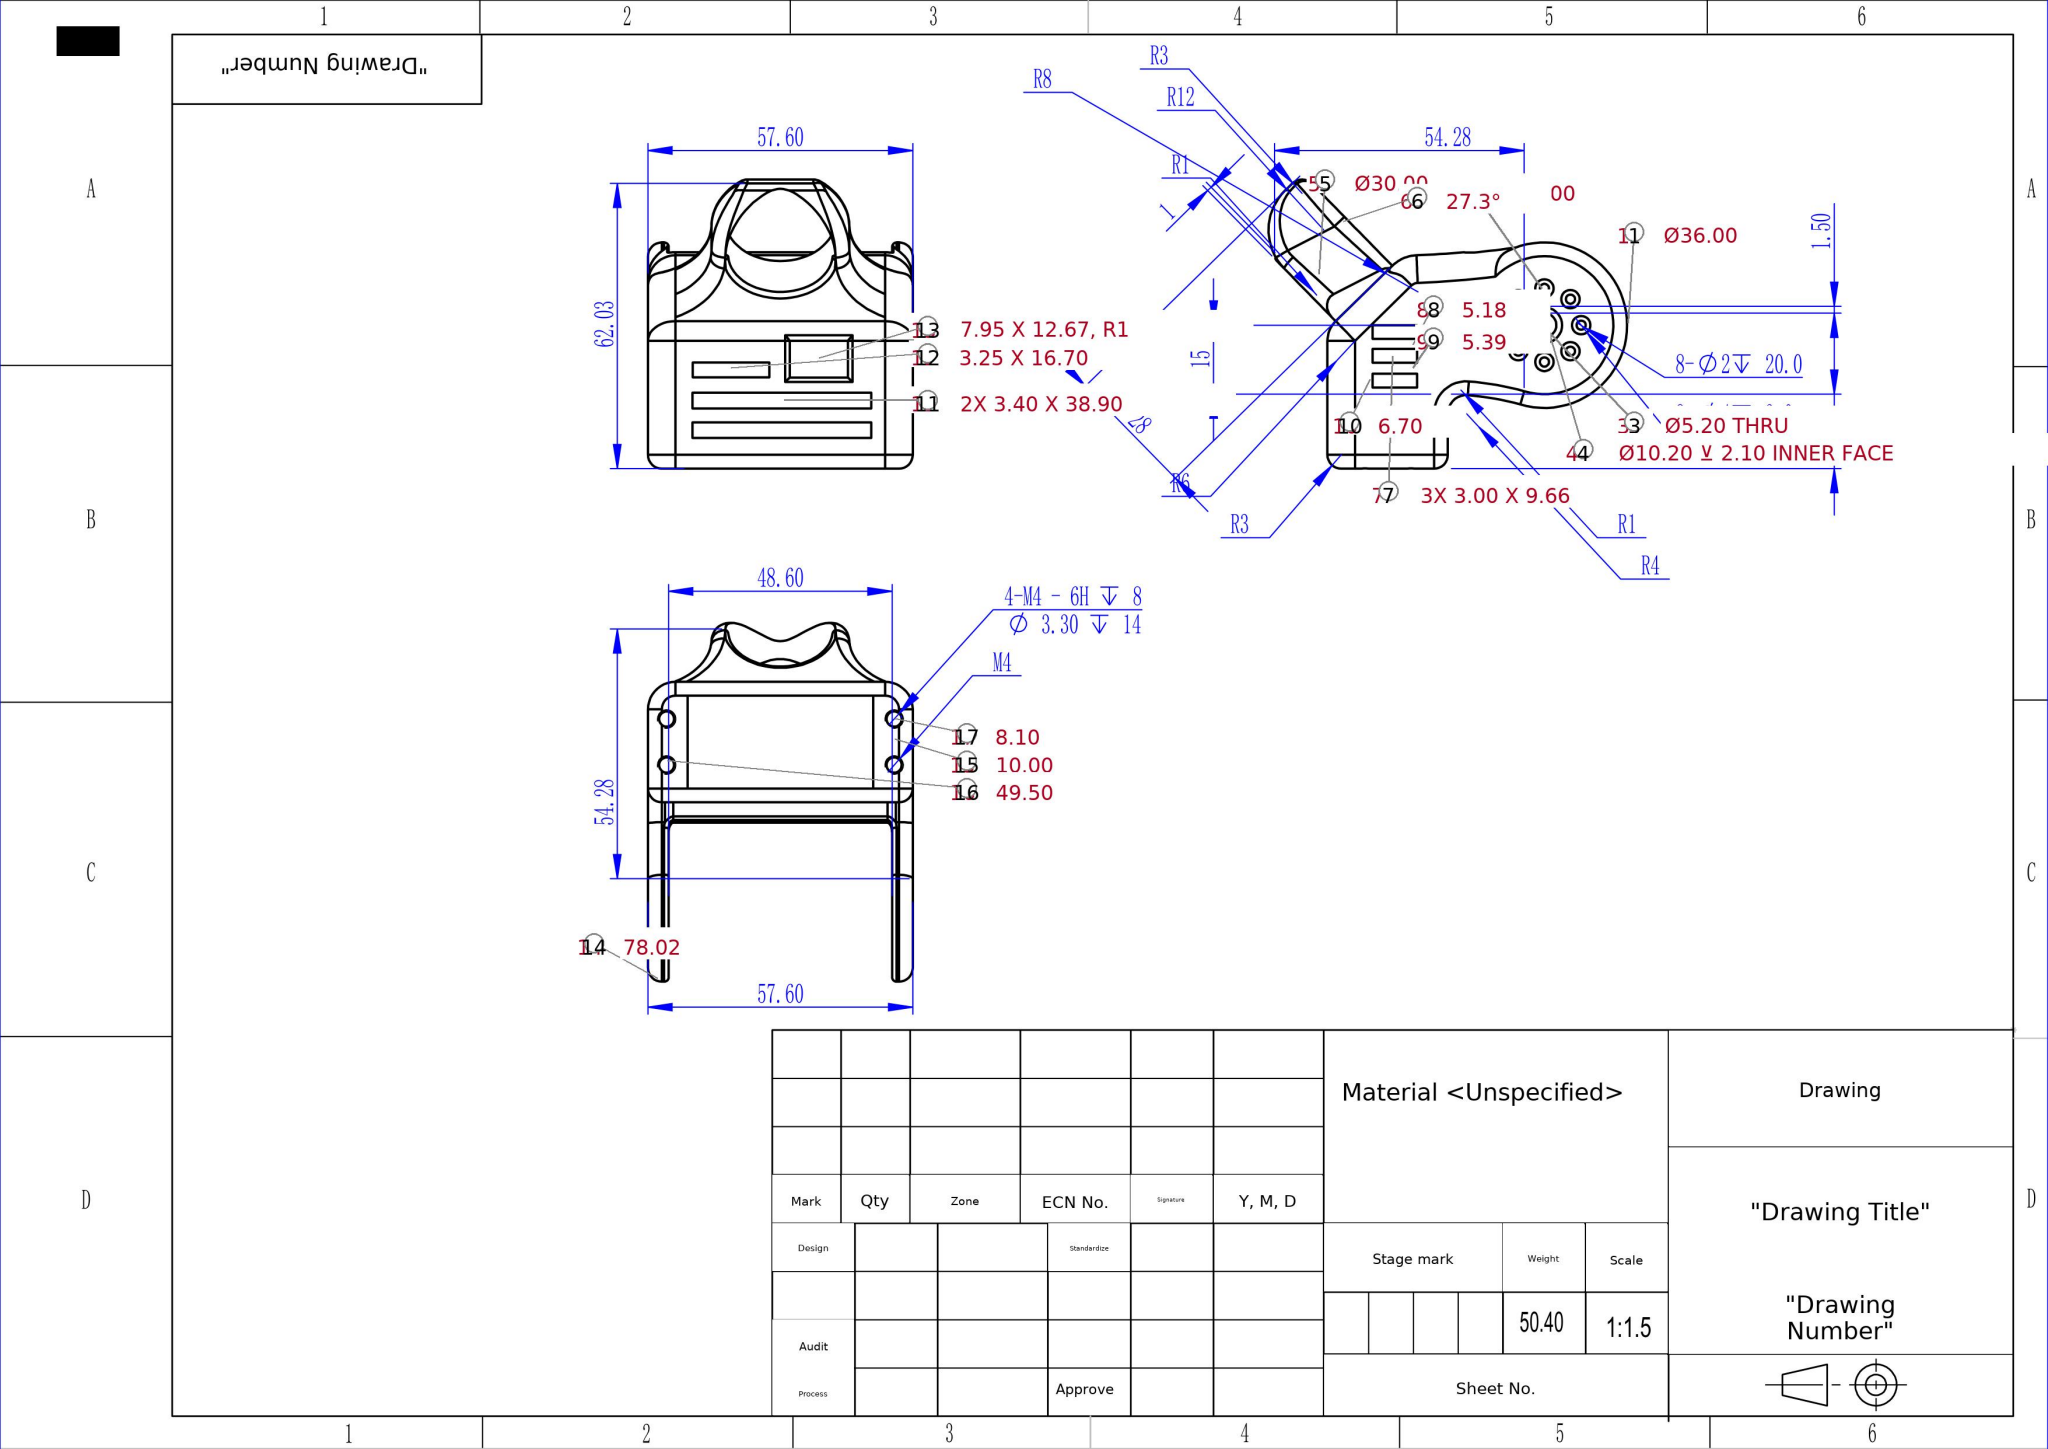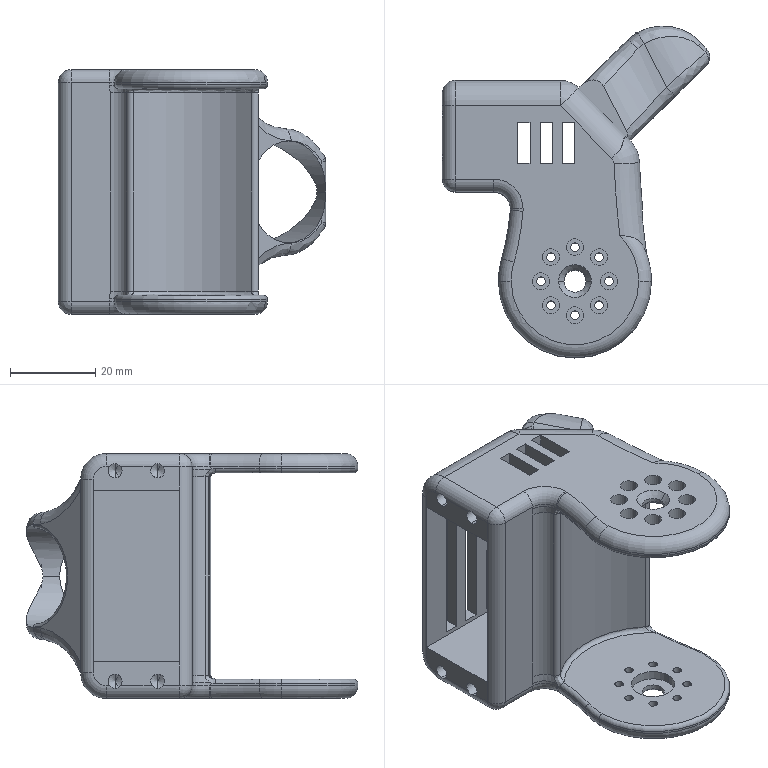Part | SolidWorks | mm | material <Unspecified> | 1 solid | 276 faces | box 62.88 x 78.02 x 57.6 mm | volume 50397 mm3 | cylinder 128 | plane 77 | torus 33 | spline 20 | cone 12 | sphere 6 | commonest cylinder face diameters 2 x39 4 x32 6 x8 3.3 x8 24 x7 36 x6 12 x5 5.2 x4